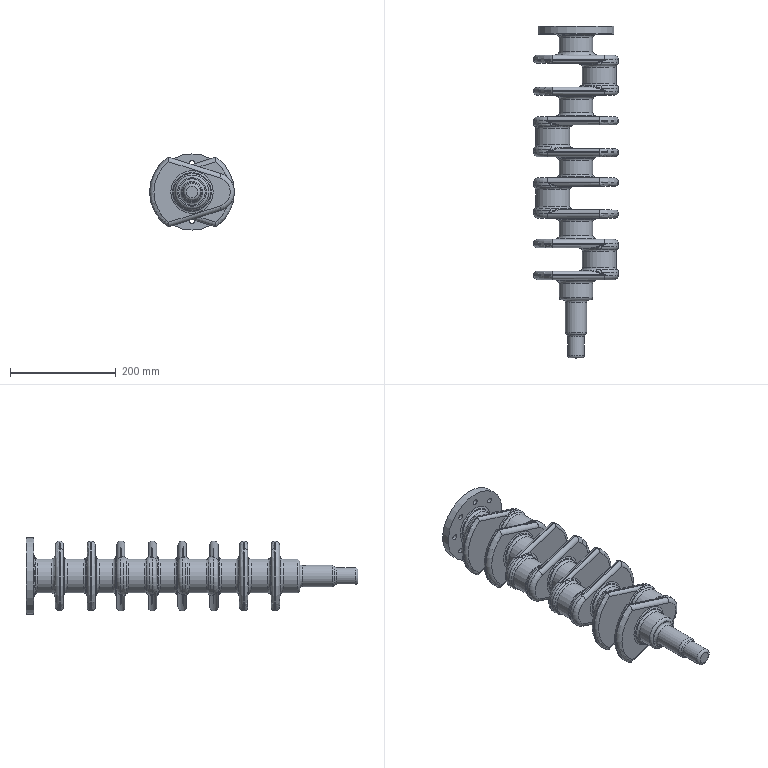Component | NX | MULTI-THROW_CRANKSHAFT | 1 solid | 255 faces | volume 3350006 mm3 | torus 87 | cylinder 68 | spline 64 | plane 36 | commonest cylinder face diameters 16 x16 12 x16 64 x9 160 x8 72 x8 10 x8 32 x1 40 x1